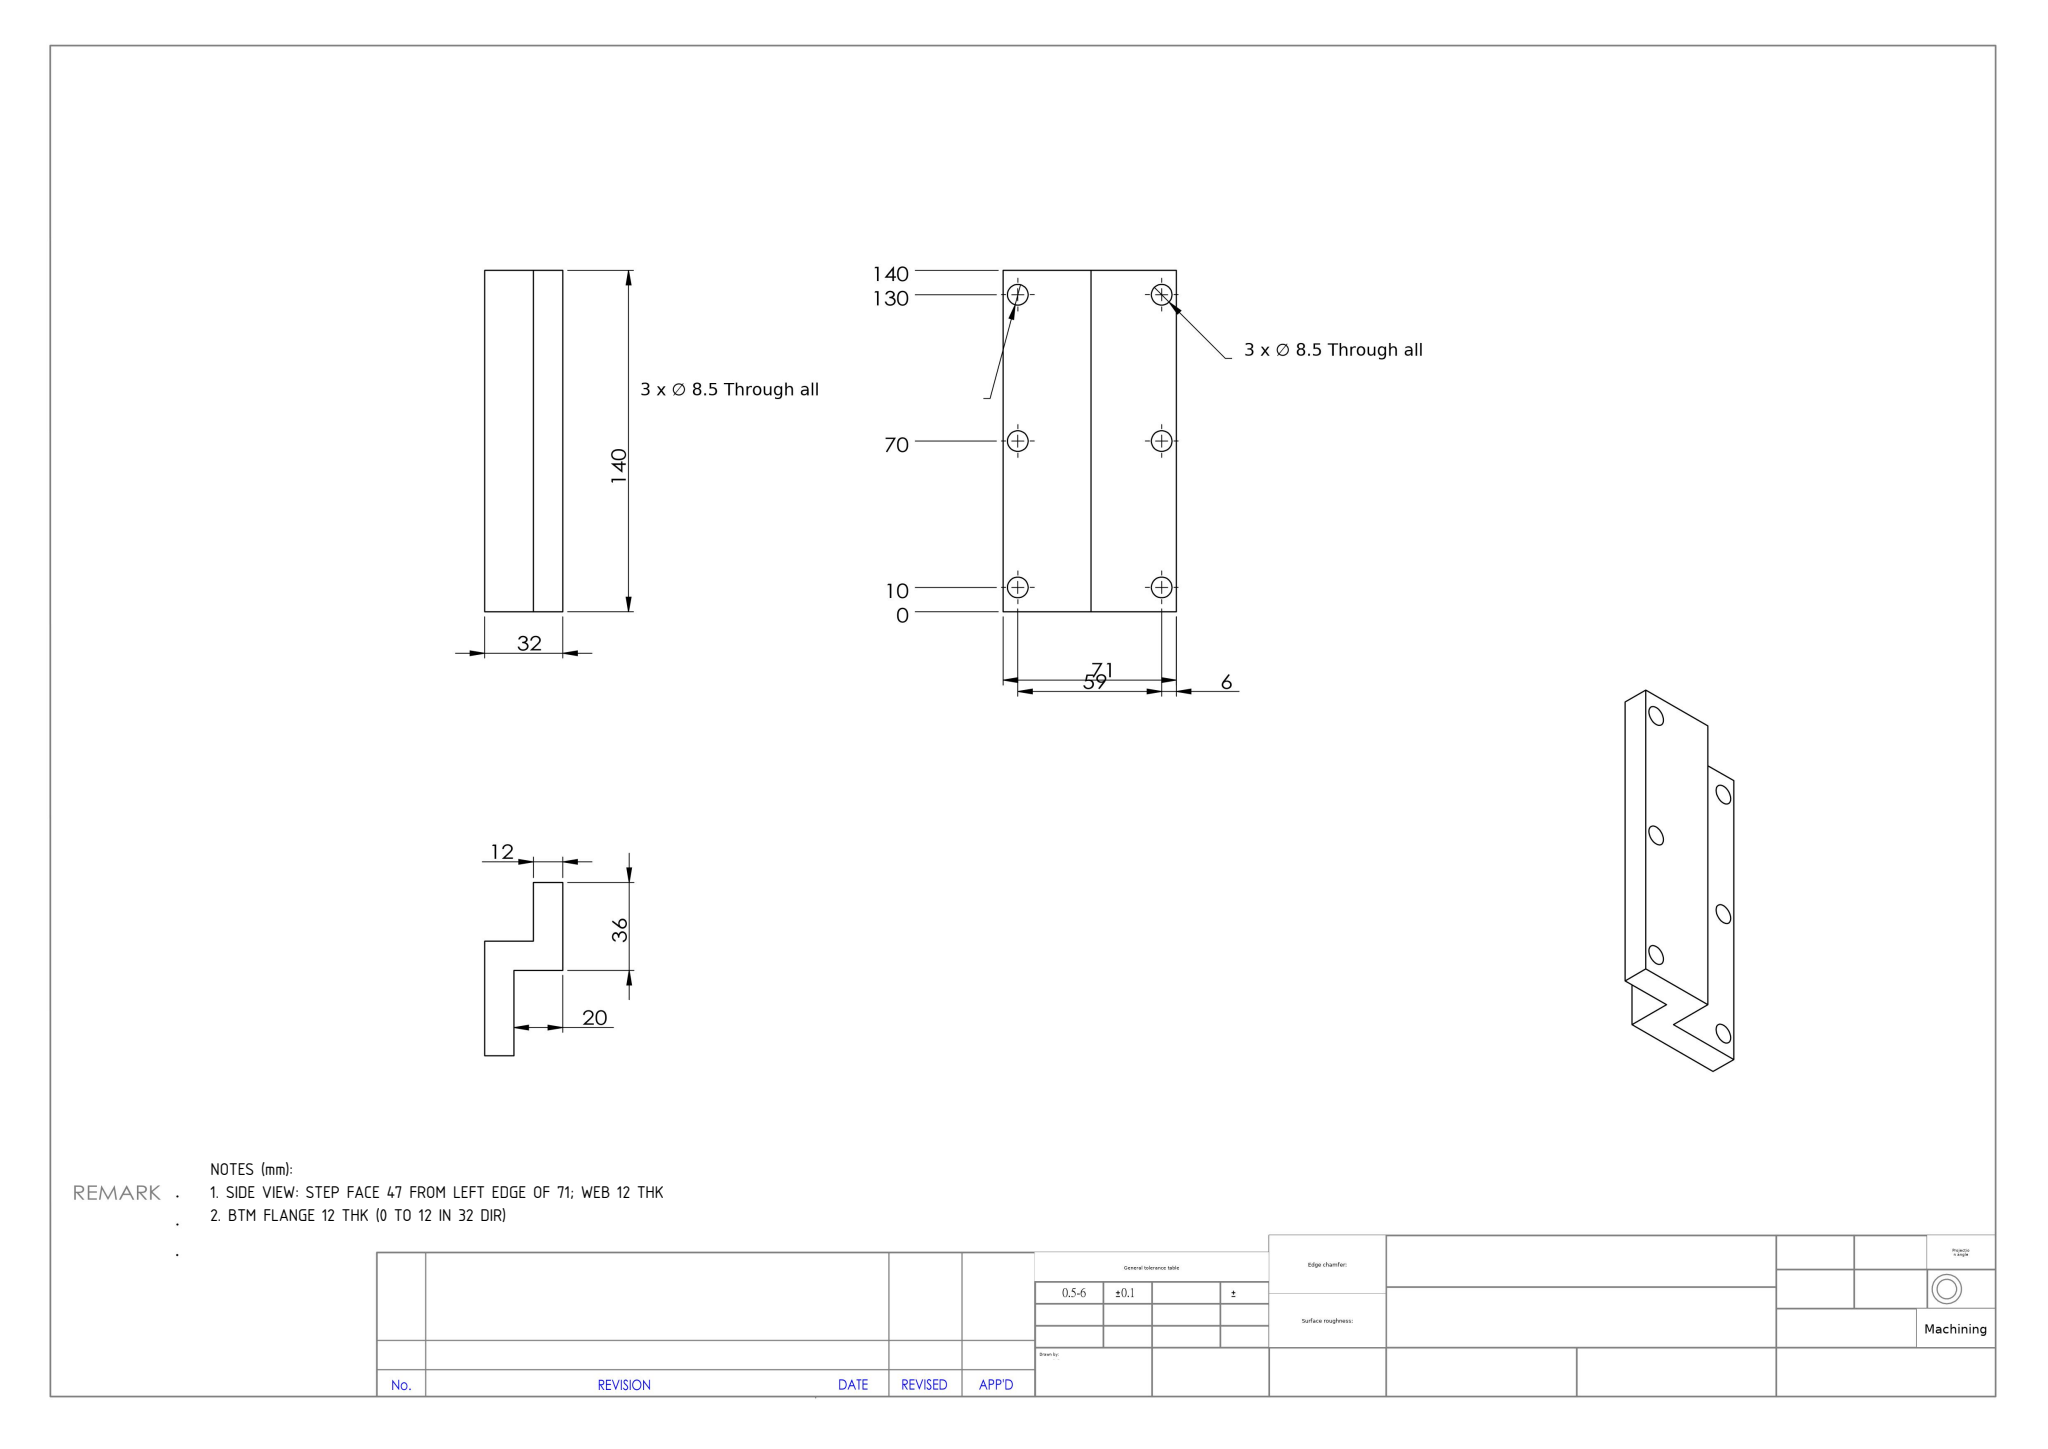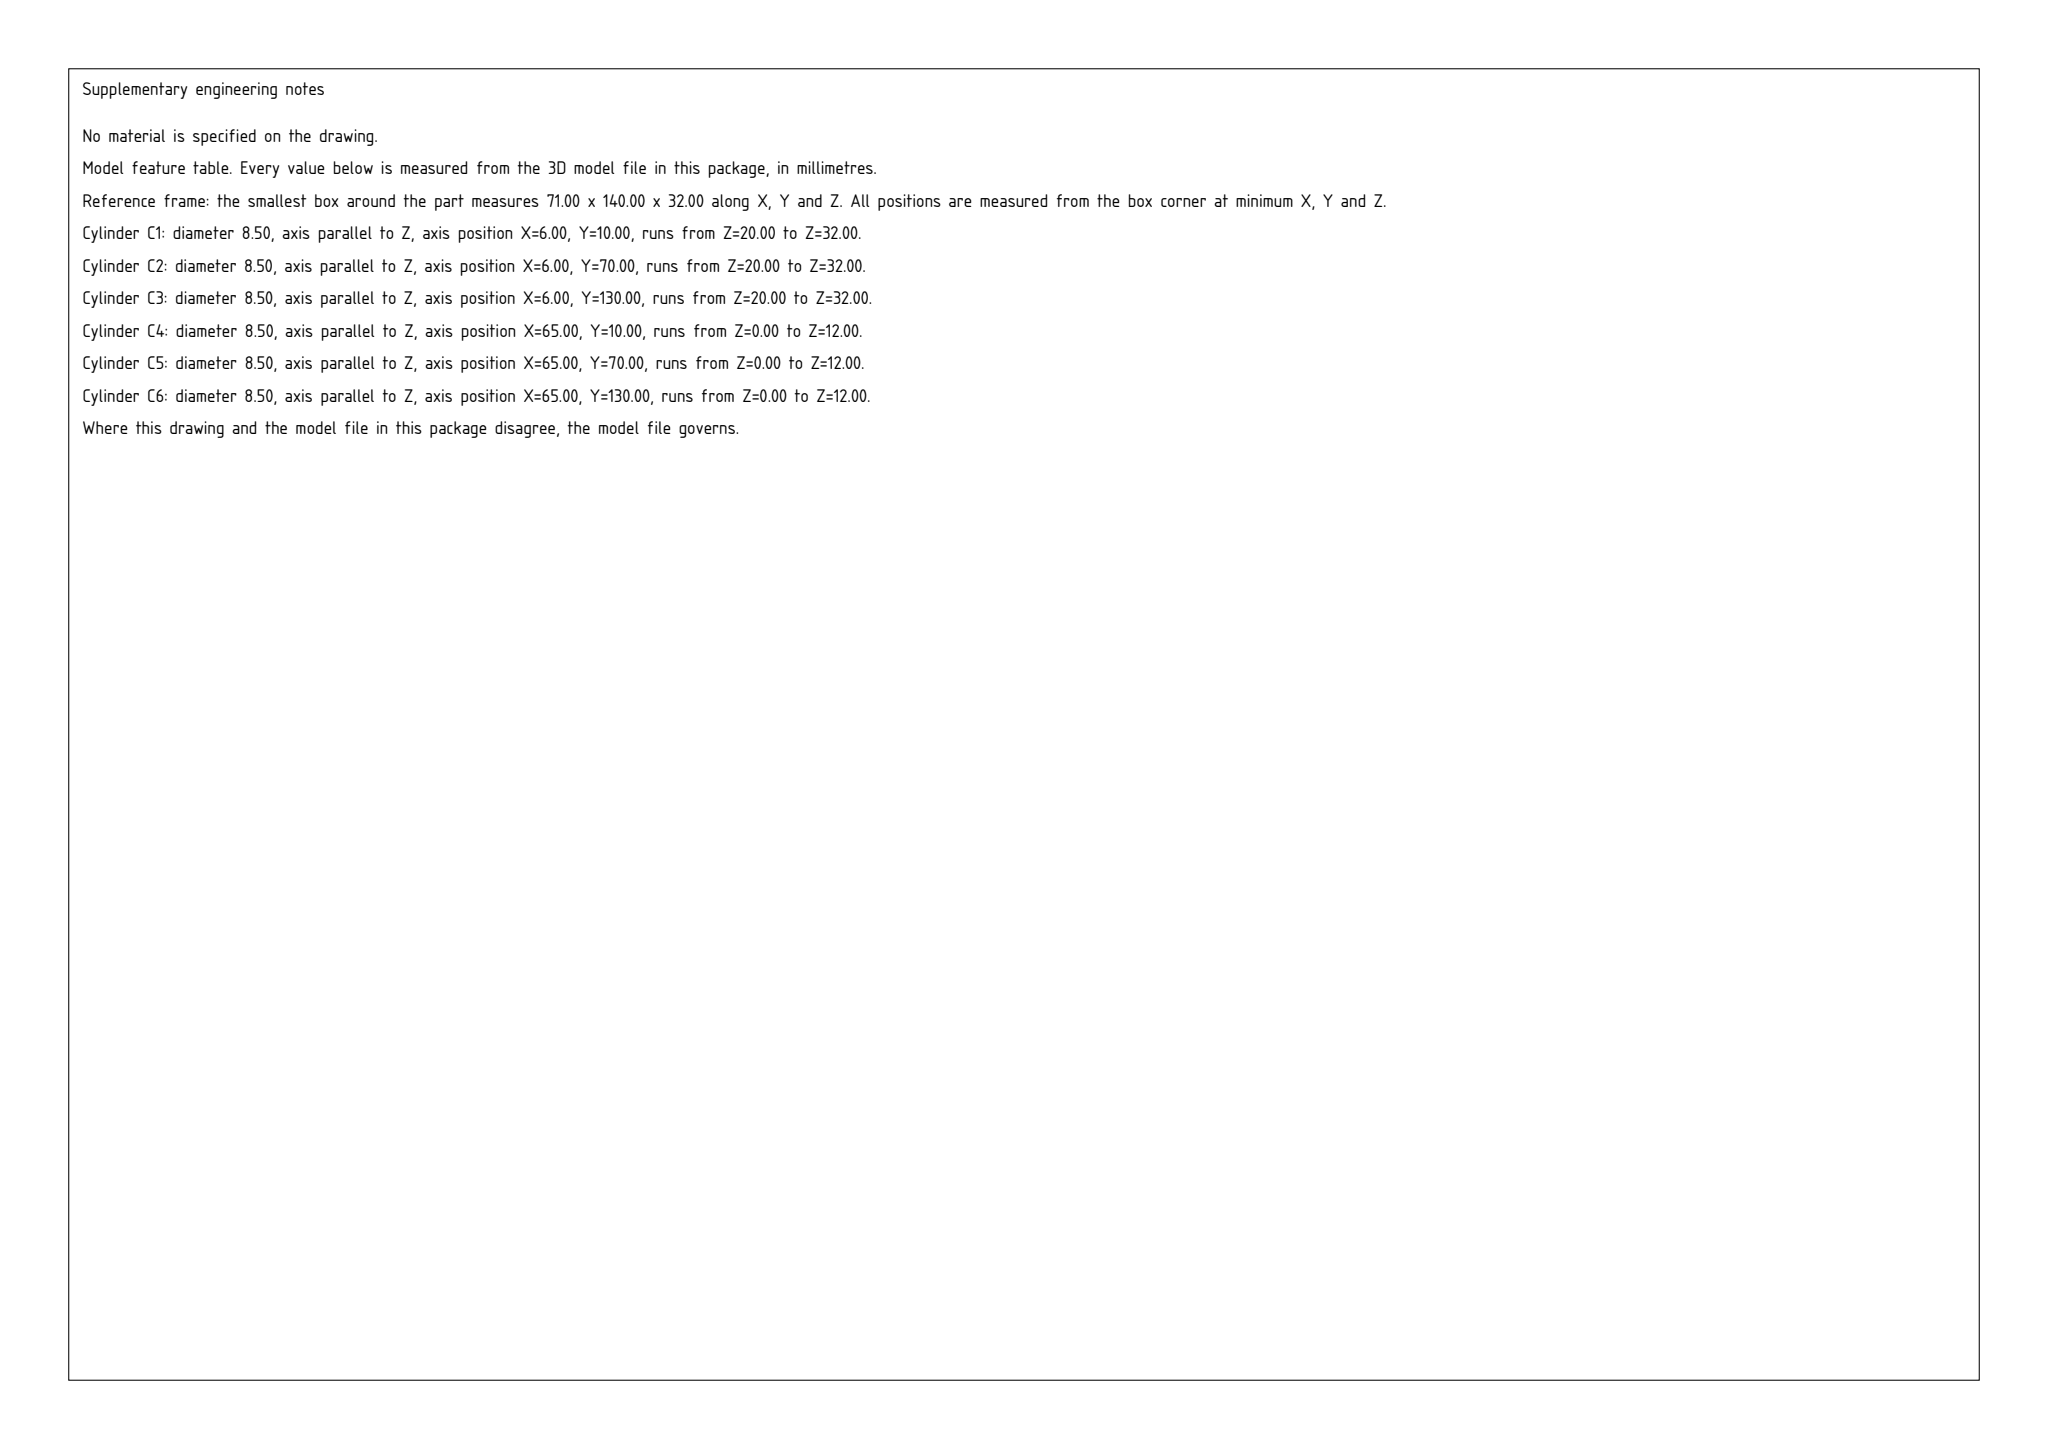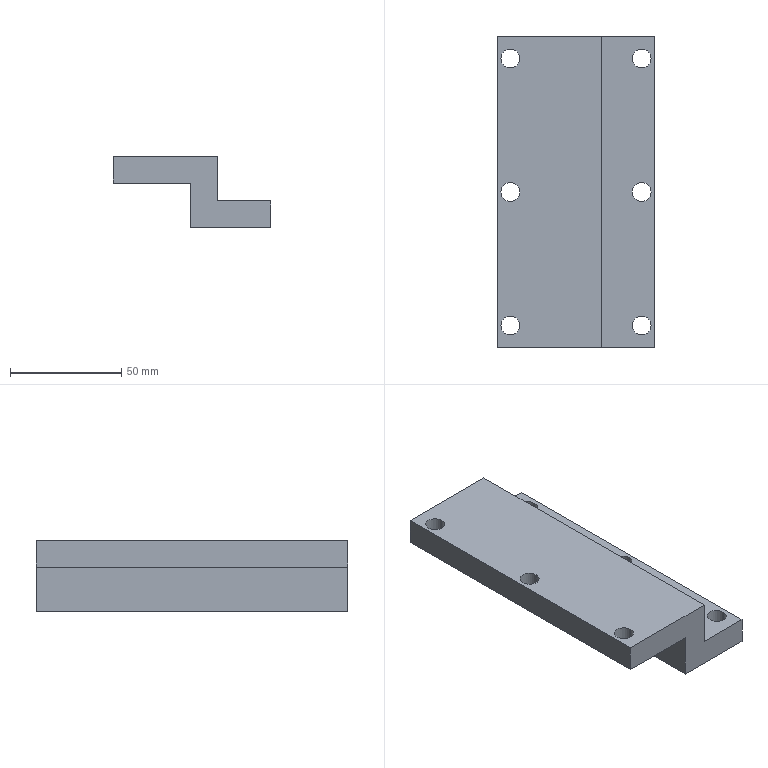Part | SolidWorks | mm | 1 solid | 22 faces | box 71 x 140 x 32 mm | volume 148794 mm3 | cylinder 12 | plane 10 | commonest cylinder face diameters 8.5 x12
Drawing notes:
SIDE VIEW: STEP FACE 47 FROM LEFT EDGE OF 71; WEB 12 THK | from the solid: axis_planes x: 0.0, 35.0, 47.0, 71.0 -> web between x35 and x47 (12 thk), lower flange face at x=47 i.e. 47 from x=0 datum used by 59/71 dims
BTM FLANGE 12 THK (0 TO 12 IN 32 DIR) | from the solid: axis_planes z: 0.0, 12.0, 20.0, 32.0 -> bottom flange spans z0-z12 = 12 thk, matching 12 upper flange and 20 step face
build123d program:
from build123d import *

# Parameters (mm, degrees)
SKETCH1_W            = 32
SKETCH1_H            = 140
BOSS_EXTRUDE1_DEPTH  = 12
SKETCH2_W            = 12
SKETCH2_H            = 140
BOSS_EXTRUDE2_DEPTH  = 24
SKETCH3_W            = 12
SKETCH3_H            = 140
BOSS_EXTRUDE3_DEPTH  = 35
M8_CLEARANCE_HOLE1_D = 8.5
M8_CLEARANCE_HOLE2_D = 8.5


with BuildPart() as part:
    # Sketch1 → Boss-Extrude1 (new body)
    with BuildSketch(Plane(origin=(0, 0, 0), x_dir=(0, 0, -1), z_dir=(1, 0, 0))):
        Rectangle(SKETCH1_W, SKETCH1_H)
    extrude(amount=BOSS_EXTRUDE1_DEPTH)

    # Sketch2 → Boss-Extrude2 (add)
    with BuildSketch(Plane(origin=(12, 0, 0), x_dir=(0, 0, -1), z_dir=(1, 0, 0))):
        with Locations((10, 0)):
            Rectangle(SKETCH2_W, SKETCH2_H)
    extrude(amount=BOSS_EXTRUDE2_DEPTH)

    # Sketch3 → Boss-Extrude3 (add)
    with BuildSketch(Plane.ZY):
        with Locations((10, 0)):
            Rectangle(SKETCH3_W, SKETCH3_H)
    extrude(amount=BOSS_EXTRUDE3_DEPTH)

    # M8 Clearance Hole1 (through all)
    with Locations(Plane(origin=(0, 0, -16), x_dir=(-1, 0, 0), z_dir=(0, 0, -1))):
        with Locations((-30, -60), (-30, 0), (-30, 60)):
            Hole(M8_CLEARANCE_HOLE1_D / 2)

    # M8 Clearance Hole2 (through all)
    with Locations(Plane(origin=(0, 0, 4), x_dir=(-1, 0, 0), z_dir=(0, 0, -1))):
        with Locations((29, 0), (29, 60), (29, -60)):
            Hole(M8_CLEARANCE_HOLE2_D / 2)


solid = part.part
STEP:
#1=CARTESIAN_POINT('',(-24.75,0.,16.));
#2=VERTEX_POINT('',#1);
#3=CARTESIAN_POINT('',(-33.25,0.,16.));
#4=VERTEX_POINT('',#3);
#5=CARTESIAN_POINT('',(-29.,0.,16.));
#6=DIRECTION('',(0.,0.,-1.));
#7=DIRECTION('',(-1.,0.,0.));
#8=AXIS2_PLACEMENT_3D('',#5,#6,#7);
#9=CIRCLE('',#8,4.25);
#10=EDGE_CURVE('',#2,#4,#9,.T.);
#11=ORIENTED_EDGE('',*,*,#10,.F.);
#12=CARTESIAN_POINT('',(-24.75,0.,4.));
#13=VERTEX_POINT('',#12);
#14=CARTESIAN_POINT('',(-24.75,0.,4.));
#15=DIRECTION('',(0.,0.,-1.));
#16=VECTOR('',#15,1000.);
#17=LINE('',#14,#16);
#18=EDGE_CURVE('',#2,#13,#17,.T.);
#19=ORIENTED_EDGE('',*,*,#18,.T.);
#20=CARTESIAN_POINT('',(-33.25,0.,4.));
#21=VERTEX_POINT('',#20);
#22=CARTESIAN_POINT('',(-29.,0.,4.));
#23=DIRECTION('',(0.,0.,-1.));
#24=DIRECTION('',(-1.,0.,0.));
#25=AXIS2_PLACEMENT_3D('',#22,#23,#24);
#26=CIRCLE('',#25,4.25);
#27=EDGE_CURVE('',#13,#21,#26,.T.);
#28=ORIENTED_EDGE('',*,*,#27,.T.);
#29=CARTESIAN_POINT('',(-33.25,0.,4.));
#30=DIRECTION('',(0.,0.,-1.));
#31=VECTOR('',#30,1000.);
#32=LINE('',#29,#31);
#33=EDGE_CURVE('',#4,#21,#32,.T.);
#34=ORIENTED_EDGE('',*,*,#33,.F.);
#35=EDGE_LOOP('',(#11,#19,#28,#34));
#36=FACE_OUTER_BOUND('',#35,.T.);
#37=CARTESIAN_POINT('',(-29.,0.,4.));
#38=DIRECTION('',(0.,0.,-1.));
#39=DIRECTION('',(-1.,0.,0.));
#40=AXIS2_PLACEMENT_3D('',#37,#38,#39);
#41=CYLINDRICAL_SURFACE('',#40,4.25);
#42=ADVANCED_FACE('',(#36),#41,.F.);
#43=CARTESIAN_POINT('',(-24.75,60.,16.));
#44=VERTEX_POINT('',#43);
#45=CARTESIAN_POINT('',(-33.25,60.,16.));
#46=VERTEX_POINT('',#45);
#47=CARTESIAN_POINT('',(-29.,60.,16.));
#48=DIRECTION('',(0.,0.,-1.));
#49=DIRECTION('',(-1.,0.,0.));
#50=AXIS2_PLACEMENT_3D('',#47,#48,#49);
#51=CIRCLE('',#50,4.25);
#52=EDGE_CURVE('',#44,#46,#51,.T.);
#53=ORIENTED_EDGE('',*,*,#52,.F.);
#54=CARTESIAN_POINT('',(-24.75,60.,4.));
#55=VERTEX_POINT('',#54);
#56=CARTESIAN_POINT('',(-24.75,60.,4.));
#57=DIRECTION('',(0.,0.,-1.));
#58=VECTOR('',#57,1000.);
#59=LINE('',#56,#58);
#60=EDGE_CURVE('',#44,#55,#59,.T.);
#61=ORIENTED_EDGE('',*,*,#60,.T.);
#62=CARTESIAN_POINT('',(-33.25,60.,4.));
#63=VERTEX_POINT('',#62);
#64=CARTESIAN_POINT('',(-29.,60.,4.));
#65=DIRECTION('',(0.,0.,-1.));
#66=DIRECTION('',(-1.,0.,0.));
#67=AXIS2_PLACEMENT_3D('',#64,#65,#66);
#68=CIRCLE('',#67,4.25);
#69=EDGE_CURVE('',#55,#63,#68,.T.);
#70=ORIENTED_EDGE('',*,*,#69,.T.);
#71=CARTESIAN_POINT('',(-33.25,60.,4.));
#72=DIRECTION('',(0.,0.,-1.));
#73=VECTOR('',#72,1000.);
#74=LINE('',#71,#73);
#75=EDGE_CURVE('',#46,#63,#74,.T.);
#76=ORIENTED_EDGE('',*,*,#75,.F.);
#77=EDGE_LOOP('',(#53,#61,#70,#76));
#78=FACE_OUTER_BOUND('',#77,.T.);
#79=CARTESIAN_POINT('',(-29.,60.,4.));
#80=DIRECTION('',(0.,0.,-1.));
#81=DIRECTION('',(-1.,0.,0.));
#82=AXIS2_PLACEMENT_3D('',#79,#80,#81);
#83=CYLINDRICAL_SURFACE('',#82,4.25);
#84=ADVANCED_FACE('',(#78),#83,.F.);
#85=CARTESIAN_POINT('',(-24.75,-60.,16.));
#86=VERTEX_POINT('',#85);
#87=CARTESIAN_POINT('',(-33.25,-60.,16.));
#88=VERTEX_POINT('',#87);
#89=CARTESIAN_POINT('',(-29.,-60.,16.));
#90=DIRECTION('',(0.,0.,-1.));
#91=DIRECTION('',(-1.,0.,0.));
#92=AXIS2_PLACEMENT_3D('',#89,#90,#91);
#93=CIRCLE('',#92,4.25);
#94=EDGE_CURVE('',#86,#88,#93,.T.);
#95=ORIENTED_EDGE('',*,*,#94,.F.);
#96=CARTESIAN_POINT('',(-24.75,-60.,4.));
#97=VERTEX_POINT('',#96);
#98=CARTESIAN_POINT('',(-24.75,-60.,4.));
#99=DIRECTION('',(0.,0.,-1.));
#100=VECTOR('',#99,1000.);
#101=LINE('',#98,#100);
#102=EDGE_CURVE('',#86,#97,#101,.T.);
#103=ORIENTED_EDGE('',*,*,#102,.T.);
#104=CARTESIAN_POINT('',(-33.25,-60.,4.));
#105=VERTEX_POINT('',#104);
#106=CARTESIAN_POINT('',(-29.,-60.,4.));
#107=DIRECTION('',(0.,0.,-1.));
#108=DIRECTION('',(-1.,0.,0.));
#109=AXIS2_PLACEMENT_3D('',#106,#107,#108);
#110=CIRCLE('',#109,4.25);
#111=EDGE_CURVE('',#97,#105,#110,.T.);
#112=ORIENTED_EDGE('',*,*,#111,.T.);
#113=CARTESIAN_POINT('',(-33.25,-60.,4.));
#114=DIRECTION('',(0.,0.,-1.));
#115=VECTOR('',#114,1000.);
#116=LINE('',#113,#115);
#117=EDGE_CURVE('',#88,#105,#116,.T.);
#118=ORIENTED_EDGE('',*,*,#117,.F.);
#119=EDGE_LOOP('',(#95,#103,#112,#118));
#120=FACE_OUTER_BOUND('',#119,.T.);
#121=CARTESIAN_POINT('',(-29.,-60.,4.));
#122=DIRECTION('',(0.,0.,-1.));
#123=DIRECTION('',(-1.,0.,0.));
#124=AXIS2_PLACEMENT_3D('',#121,#122,#123);
#125=CYLINDRICAL_SURFACE('',#124,4.25);
#126=ADVANCED_FACE('',(#120),#125,.F.);
#127=CARTESIAN_POINT('',(34.25,0.,-4.));
#128=VERTEX_POINT('',#127);
#129=CARTESIAN_POINT('',(25.75,0.,-4.));
#130=VERTEX_POINT('',#129);
#131=CARTESIAN_POINT('',(30.,0.,-4.));
#132=DIRECTION('',(0.,0.,-1.));
#133=DIRECTION('',(0.,1.,0.));
#134=AXIS2_PLACEMENT_3D('',#131,#132,#133);
#135=CIRCLE('',#134,4.25);
#136=EDGE_CURVE('',#128,#130,#135,.T.);
#137=ORIENTED_EDGE('',*,*,#136,.F.);
#138=CARTESIAN_POINT('',(34.25,0.,-16.));
#139=VERTEX_POINT('',#138);
#140=CARTESIAN_POINT('',(34.25,0.,-16.));
#141=DIRECTION('',(0.,0.,-1.));
#142=VECTOR('',#141,1000.);
#143=LINE('',#140,#142);
#144=EDGE_CURVE('',#128,#139,#143,.T.);
#145=ORIENTED_EDGE('',*,*,#144,.T.);
#146=CARTESIAN_POINT('',(25.75,0.,-16.));
#147=VERTEX_POINT('',#146);
#148=CARTESIAN_POINT('',(30.,0.,-16.));
#149=DIRECTION('',(0.,0.,-1.));
#150=DIRECTION('',(-1.,0.,0.));
#151=AXIS2_PLACEMENT_3D('',#148,#149,#150);
#152=CIRCLE('',#151,4.25);
#153=EDGE_CURVE('',#139,#147,#152,.T.);
#154=ORIENTED_EDGE('',*,*,#153,.T.);
#155=CARTESIAN_POINT('',(25.75,0.,-16.));
#156=DIRECTION('',(0.,0.,-1.));
#157=VECTOR('',#156,1000.);
#158=LINE('',#155,#157);
#159=EDGE_CURVE('',#130,#147,#158,.T.);
#160=ORIENTED_EDGE('',*,*,#159,.F.);
#161=EDGE_LOOP('',(#137,#145,#154,#160));
#162=FACE_OUTER_BOUND('',#161,.T.);
#163=CARTESIAN_POINT('',(30.,0.,-16.));
#164=DIRECTION('',(0.,0.,-1.));
#165=DIRECTION('',(-1.,0.,0.));
#166=AXIS2_PLACEMENT_3D('',#163,#164,#165);
#167=CYLINDRICAL_SURFACE('',#166,4.25);
#168=ADVANCED_FACE('',(#162),#167,.F.);
#169=CARTESIAN_POINT('',(34.25,60.,-4.));
#170=VERTEX_POINT('',#169);
#171=CARTESIAN_POINT('',(25.75,60.,-4.));
#172=VERTEX_POINT('',#171);
#173=CARTESIAN_POINT('',(30.,60.,-4.));
#174=DIRECTION('',(0.,0.,-1.));
#175=DIRECTION('',(0.,1.,0.));
#176=AXIS2_PLACEMENT_3D('',#173,#174,#175);
#177=CIRCLE('',#176,4.25);
#178=EDGE_CURVE('',#170,#172,#177,.T.);
#179=ORIENTED_EDGE('',*,*,#178,.F.);
#180=CARTESIAN_POINT('',(34.25,60.,-16.));
#181=VERTEX_POINT('',#180);
#182=CARTESIAN_POINT('',(34.25,60.,-16.));
#183=DIRECTION('',(0.,0.,-1.));
#184=VECTOR('',#183,1000.);
#185=LINE('',#182,#184);
#186=EDGE_CURVE('',#170,#181,#185,.T.);
#187=ORIENTED_EDGE('',*,*,#186,.T.);
#188=CARTESIAN_POINT('',(25.75,60.,-16.));
#189=VERTEX_POINT('',#188);
#190=CARTESIAN_POINT('',(30.,60.,-16.));
#191=DIRECTION('',(0.,0.,-1.));
#192=DIRECTION('',(-1.,0.,0.));
#193=AXIS2_PLACEMENT_3D('',#190,#191,#192);
#194=CIRCLE('',#193,4.25);
#195=EDGE_CURVE('',#181,#189,#194,.T.);
#196=ORIENTED_EDGE('',*,*,#195,.T.);
#197=CARTESIAN_POINT('',(25.75,60.,-16.));
#198=DIRECTION('',(0.,0.,-1.));
#199=VECTOR('',#198,1000.);
#200=LINE('',#197,#199);
#201=EDGE_CURVE('',#172,#189,#200,.T.);
#202=ORIENTED_EDGE('',*,*,#201,.F.);
#203=EDGE_LOOP('',(#179,#187,#196,#202));
#204=FACE_OUTER_BOUND('',#203,.T.);
#205=CARTESIAN_POINT('',(30.,60.,-16.));
#206=DIRECTION('',(0.,0.,-1.));
#207=DIRECTION('',(-1.,0.,0.));
#208=AXIS2_PLACEMENT_3D('',#205,#206,#207);
#209=CYLINDRICAL_SURFACE('',#208,4.25);
#210=ADVANCED_FACE('',(#204),#209,.F.);
#211=CARTESIAN_POINT('',(34.25,-60.,-4.));
#212=VERTEX_POINT('',#211);
#213=CARTESIAN_POINT('',(25.75,-60.,-4.));
#214=VERTEX_POINT('',#213);
#215=CARTESIAN_POINT('',(30.,-60.,-4.));
#216=DIRECTION('',(0.,0.,-1.));
#217=DIRECTION('',(0.,1.,0.));
#218=AXIS2_PLACEMENT_3D('',#215,#216,#217);
#219=CIRCLE('',#218,4.25);
#220=EDGE_CURVE('',#212,#214,#219,.T.);
#221=ORIENTED_EDGE('',*,*,#220,.F.);
#222=CARTESIAN_POINT('',(34.25,-60.,-16.));
#223=VERTEX_POINT('',#222);
#224=CARTESIAN_POINT('',(34.25,-60.,-16.));
#225=DIRECTION('',(0.,0.,-1.));
#226=VECTOR('',#225,1000.);
#227=LINE('',#224,#226);
#228=EDGE_CURVE('',#212,#223,#227,.T.);
#229=ORIENTED_EDGE('',*,*,#228,.T.);
#230=CARTESIAN_POINT('',(25.75,-60.,-16.));
#231=VERTEX_POINT('',#230);
#232=CARTESIAN_POINT('',(30.,-60.,-16.));
#233=DIRECTION('',(0.,0.,-1.));
#234=DIRECTION('',(-1.,0.,0.));
#235=AXIS2_PLACEMENT_3D('',#232,#233,#234);
#236=CIRCLE('',#235,4.25);
#237=EDGE_CURVE('',#223,#231,#236,.T.);
#238=ORIENTED_EDGE('',*,*,#237,.T.);
#239=CARTESIAN_POINT('',(25.75,-60.,-16.));
#240=DIRECTION('',(0.,0.,-1.));
#241=VECTOR('',#240,1000.);
#242=LINE('',#239,#241);
#243=EDGE_CURVE('',#214,#231,#242,.T.);
#244=ORIENTED_EDGE('',*,*,#243,.F.);
#245=EDGE_LOOP('',(#221,#229,#238,#244));
#246=FACE_OUTER_BOUND('',#245,.T.);
#247=CARTESIAN_POINT('',(30.,-60.,-16.));
#248=DIRECTION('',(0.,0.,-1.));
#249=DIRECTION('',(-1.,0.,0.));
#250=AXIS2_PLACEMENT_3D('',#247,#248,#249);
#251=CYLINDRICAL_SURFACE('',#250,4.25);
#252=ADVANCED_FACE('',(#246),#251,.F.);
#253=CARTESIAN_POINT('',(12.,70.,-4.));
#254=VERTEX_POINT('',#253);
#255=CARTESIAN_POINT('',(12.,-70.,-4.));
#256=VERTEX_POINT('',#255);
#257=CARTESIAN_POINT('',(12.,70.,-4.));
#258=DIRECTION('',(0.,-1.,-0.));
#259=VECTOR('',#258,1000.);
#260=LINE('',#257,#259);
#261=EDGE_CURVE('',#254,#256,#260,.T.);
#262=ORIENTED_EDGE('',*,*,#261,.F.);
#263=CARTESIAN_POINT('',(12.,70.,16.));
#264=VERTEX_POINT('',#263);
#265=CARTESIAN_POINT('',(12.,70.,16.));
#266=DIRECTION('',(0.,0.,1.));
#267=VECTOR('',#266,1000.);
#268=LINE('',#265,#267);
#269=EDGE_CURVE('',#254,#264,#268,.T.);
#270=ORIENTED_EDGE('',*,*,#269,.T.);
#271=CARTESIAN_POINT('',(12.,-70.,16.));
#272=VERTEX_POINT('',#271);
#273=CARTESIAN_POINT('',(12.,-70.,16.));
#274=DIRECTION('',(0.,-1.,0.));
#275=VECTOR('',#274,1000.);
#276=LINE('',#273,#275);
#277=EDGE_CURVE('',#264,#272,#276,.T.);
#278=ORIENTED_EDGE('',*,*,#277,.T.);
#279=CARTESIAN_POINT('',(12.,-70.,16.));
#280=DIRECTION('',(0.,0.,-1.));
#281=VECTOR('',#280,1000.);
#282=LINE('',#279,#281);
#283=EDGE_CURVE('',#272,#256,#282,.T.);
#284=ORIENTED_EDGE('',*,*,#283,.T.);
#285=EDGE_LOOP('',(#262,#270,#278,#284));
#286=FACE_OUTER_BOUND('',#285,.T.);
#287=CARTESIAN_POINT('',(12.,0.,0.));
#288=DIRECTION('',(-1.,0.,0.));
#289=DIRECTION('',(0.,0.,1.));
#290=AXIS2_PLACEMENT_3D('',#287,#288,#289);
#291=PLANE('',#290);
#292=ADVANCED_FACE('',(#286),#291,.F.);
#293=CARTESIAN_POINT('',(30.,0.,-16.));
#294=DIRECTION('',(0.,0.,-1.));
#295=DIRECTION('',(-1.,0.,0.));
#296=AXIS2_PLACEMENT_3D('',#293,#294,#295);
#297=CIRCLE('',#296,4.25);
#298=EDGE_CURVE('',#147,#139,#297,.T.);
#299=ORIENTED_EDGE('',*,*,#298,.F.);
#300=ORIENTED_EDGE('',*,*,#153,.F.);
#301=EDGE_LOOP('',(#299,#300));
#302=FACE_BOUND('',#301,.T.);
#303=CARTESIAN_POINT('',(30.,60.,-16.));
#304=DIRECTION('',(0.,0.,-1.));
#305=DIRECTION('',(-1.,0.,0.));
#306=AXIS2_PLACEMENT_3D('',#303,#304,#305);
#307=CIRCLE('',#306,4.25);
#308=EDGE_CURVE('',#189,#181,#307,.T.);
#309=ORIENTED_EDGE('',*,*,#308,.F.);
#310=ORIENTED_EDGE('',*,*,#195,.F.);
#311=EDGE_LOOP('',(#309,#310));
#312=FACE_BOUND('',#311,.T.);
#313=CARTESIAN_POINT('',(30.,-60.,-16.));
#314=DIRECTION('',(0.,0.,-1.));
#315=DIRECTION('',(-1.,0.,0.));
#316=AXIS2_PLACEMENT_3D('',#313,#314,#315);
#317=CIRCLE('',#316,4.25);
#318=EDGE_CURVE('',#231,#223,#317,.T.);
#319=ORIENTED_EDGE('',*,*,#318,.F.);
#320=ORIENTED_EDGE('',*,*,#237,.F.);
#321=EDGE_LOOP('',(#319,#320));
#322=FACE_BOUND('',#321,.T.);
#323=CARTESIAN_POINT('',(0.,-70.,-16.));
#324=VERTEX_POINT('',#323);
#325=CARTESIAN_POINT('',(0.,70.,-16.));
#326=VERTEX_POINT('',#325);
#327=CARTESIAN_POINT('',(0.,-70.,-16.));
#328=DIRECTION('',(0.,1.,0.));
#329=VECTOR('',#328,1000.);
#330=LINE('',#327,#329);
#331=EDGE_CURVE('',#324,#326,#330,.T.);
#332=ORIENTED_EDGE('',*,*,#331,.T.);
#333=CARTESIAN_POINT('',(36.,70.,-16.));
#334=VERTEX_POINT('',#333);
#335=CARTESIAN_POINT('',(12.,70.,-16.));
#336=DIRECTION('',(-1.,0.,0.));
#337=VECTOR('',#336,1000.);
#338=LINE('',#335,#337);
#339=EDGE_CURVE('',#334,#326,#338,.T.);
#340=ORIENTED_EDGE('',*,*,#339,.F.);
#341=CARTESIAN_POINT('',(36.,-70.,-16.));
#342=VERTEX_POINT('',#341);
#343=CARTESIAN_POINT('',(36.,70.,-16.));
#344=DIRECTION('',(0.,1.,0.));
#345=VECTOR('',#344,1000.);
#346=LINE('',#343,#345);
#347=EDGE_CURVE('',#342,#334,#346,.T.);
#348=ORIENTED_EDGE('',*,*,#347,.F.);
#349=CARTESIAN_POINT('',(12.,-70.,-16.));
#350=DIRECTION('',(-1.,0.,0.));
#351=VECTOR('',#350,1000.);
#352=LINE('',#349,#351);
#353=EDGE_CURVE('',#342,#324,#352,.T.);
#354=ORIENTED_EDGE('',*,*,#353,.T.);
#355=EDGE_LOOP('',(#332,#340,#348,#354));
#356=FACE_OUTER_BOUND('',#355,.T.);
#357=CARTESIAN_POINT('',(12.,-70.,-16.));
#358=DIRECTION('',(0.,0.,1.));
#359=DIRECTION('',(1.,0.,0.));
#360=AXIS2_PLACEMENT_3D('',#357,#358,#359);
#361=PLANE('',#360);
#362=ADVANCED_FACE('',(#302,#312,#322,#356),#361,.F.);
#363=CARTESIAN_POINT('',(0.,70.,4.));
#364=VERTEX_POINT('',#363);
#365=CARTESIAN_POINT('',(0.,70.,16.));
#366=DIRECTION('',(0.,0.,1.));
#367=VECTOR('',#366,1000.);
#368=LINE('',#365,#367);
#369=EDGE_CURVE('',#326,#364,#368,.T.);
#370=ORIENTED_EDGE('',*,*,#369,.T.);
#371=CARTESIAN_POINT('',(-35.,70.,4.));
#372=VERTEX_POINT('',#371);
#373=CARTESIAN_POINT('',(-35.,70.,4.));
#374=DIRECTION('',(1.,0.,0.));
#375=VECTOR('',#374,1000.);
#376=LINE('',#373,#375);
#377=EDGE_CURVE('',#372,#364,#376,.T.);
#378=ORIENTED_EDGE('',*,*,#377,.F.);
#379=CARTESIAN_POINT('',(-35.,70.,16.));
#380=VERTEX_POINT('',#379);
#381=CARTESIAN_POINT('',(-35.,70.,16.));
#382=DIRECTION('',(0.,0.,-1.));
#383=VECTOR('',#382,1000.);
#384=LINE('',#381,#383);
#385=EDGE_CURVE('',#380,#372,#384,.T.);
#386=ORIENTED_EDGE('',*,*,#385,.F.);
#387=CARTESIAN_POINT('',(12.,70.,16.));
#388=DIRECTION('',(-1.,0.,0.));
#389=VECTOR('',#388,1000.);
#390=LINE('',#387,#389);
#391=EDGE_CURVE('',#264,#380,#390,.T.);
#392=ORIENTED_EDGE('',*,*,#391,.F.);
#393=ORIENTED_EDGE('',*,*,#269,.F.);
#394=CARTESIAN_POINT('',(36.,70.,-4.));
#395=VERTEX_POINT('',#394);
#396=CARTESIAN_POINT('',(36.,70.,-4.));
#397=DIRECTION('',(-1.,0.,0.));
#398=VECTOR('',#397,1000.);
#399=LINE('',#396,#398);
#400=EDGE_CURVE('',#395,#254,#399,.T.);
#401=ORIENTED_EDGE('',*,*,#400,.F.);
#402=CARTESIAN_POINT('',(36.,70.,-16.));
#403=DIRECTION('',(0.,0.,1.));
#404=VECTOR('',#403,1000.);
#405=LINE('',#402,#404);
#406=EDGE_CURVE('',#334,#395,#405,.T.);
#407=ORIENTED_EDGE('',*,*,#406,.F.);
#408=ORIENTED_EDGE('',*,*,#339,.T.);
#409=EDGE_LOOP('',(#370,#378,#386,#392,#393,#401,#407,#408));
#410=FACE_OUTER_BOUND('',#409,.T.);
#411=CARTESIAN_POINT('',(12.,70.,16.));
#412=DIRECTION('',(0.,-1.,0.));
#413=DIRECTION('',(0.,0.,-1.));
#414=AXIS2_PLACEMENT_3D('',#411,#412,#413);
#415=PLANE('',#414);
#416=ADVANCED_FACE('',(#410),#415,.F.);
#417=CARTESIAN_POINT('',(-29.,0.,16.));
#418=DIRECTION('',(0.,0.,-1.));
#419=DIRECTION('',(-1.,0.,0.));
#420=AXIS2_PLACEMENT_3D('',#417,#418,#419);
#421=CIRCLE('',#420,4.25);
#422=EDGE_CURVE('',#4,#2,#421,.T.);
#423=ORIENTED_EDGE('',*,*,#422,.T.);
#424=ORIENTED_EDGE('',*,*,#10,.T.);
#425=EDGE_LOOP('',(#423,#424));
#426=FACE_BOUND('',#425,.T.);
#427=CARTESIAN_POINT('',(-29.,60.,16.));
#428=DIRECTION('',(0.,0.,-1.));
#429=DIRECTION('',(-1.,0.,0.));
#430=AXIS2_PLACEMENT_3D('',#427,#428,#429);
#431=CIRCLE('',#430,4.25);
#432=EDGE_CURVE('',#46,#44,#431,.T.);
#433=ORIENTED_EDGE('',*,*,#432,.T.);
#434=ORIENTED_EDGE('',*,*,#52,.T.);
#435=EDGE_LOOP('',(#433,#434));
#436=FACE_BOUND('',#435,.T.);
#437=CARTESIAN_POINT('',(-29.,-60.,16.));
#438=DIRECTION('',(0.,0.,-1.));
#439=DIRECTION('',(-1.,0.,0.));
#440=AXIS2_PLACEMENT_3D('',#437,#438,#439);
#441=CIRCLE('',#440,4.25);
#442=EDGE_CURVE('',#88,#86,#441,.T.);
#443=ORIENTED_EDGE('',*,*,#442,.T.);
#444=ORIENTED_EDGE('',*,*,#94,.T.);
#445=EDGE_LOOP('',(#443,#444));
#446=FACE_BOUND('',#445,.T.);
#447=ORIENTED_EDGE('',*,*,#391,.T.);
#448=CARTESIAN_POINT('',(-35.,-70.,16.));
#449=VERTEX_POINT('',#448);
#450=CARTESIAN_POINT('',(-35.,-70.,16.));
#451=DIRECTION('',(0.,1.,0.));
#452=VECTOR('',#451,1000.);
#453=LINE('',#450,#452);
#454=EDGE_CURVE('',#449,#380,#453,.T.);
#455=ORIENTED_EDGE('',*,*,#454,.F.);
#456=CARTESIAN_POINT('',(12.,-70.,16.));
#457=DIRECTION('',(-1.,0.,0.));
#458=VECTOR('',#457,1000.);
#459=LINE('',#456,#458);
#460=EDGE_CURVE('',#272,#449,#459,.T.);
#461=ORIENTED_EDGE('',*,*,#460,.F.);
#462=ORIENTED_EDGE('',*,*,#277,.F.);
#463=EDGE_LOOP('',(#447,#455,#461,#462));
#464=FACE_OUTER_BOUND('',#463,.T.);
#465=CARTESIAN_POINT('',(12.,-70.,16.));
#466=DIRECTION('',(0.,0.,-1.));
#467=DIRECTION('',(-1.,0.,0.));
#468=AXIS2_PLACEMENT_3D('',#465,#466,#467);
#469=PLANE('',#468);
#470=ADVANCED_FACE('',(#426,#436,#446,#464),#469,.F.);
#471=ORIENTED_EDGE('',*,*,#460,.T.);
#472=CARTESIAN_POINT('',(-35.,-70.,4.));
#473=VERTEX_POINT('',#472);
#474=CARTESIAN_POINT('',(-35.,-70.,16.));
#475=DIRECTION('',(0.,0.,1.));
#476=VECTOR('',#475,1000.);
#477=LINE('',#474,#476);
#478=EDGE_CURVE('',#473,#449,#477,.T.);
#479=ORIENTED_EDGE('',*,*,#478,.F.);
#480=CARTESIAN_POINT('',(0.,-70.,4.));
#481=VERTEX_POINT('',#480);
#482=CARTESIAN_POINT('',(-35.,-70.,4.));
#483=DIRECTION('',(1.,0.,0.));
#484=VECTOR('',#483,1000.);
#485=LINE('',#482,#484);
#486=EDGE_CURVE('',#473,#481,#485,.T.);
#487=ORIENTED_EDGE('',*,*,#486,.T.);
#488=CARTESIAN_POINT('',(0.,-70.,16.));
#489=DIRECTION('',(0.,0.,-1.));
#490=VECTOR('',#489,1000.);
#491=LINE('',#488,#490);
#492=EDGE_CURVE('',#481,#324,#491,.T.);
#493=ORIENTED_EDGE('',*,*,#492,.T.);
#494=ORIENTED_EDGE('',*,*,#353,.F.);
#495=CARTESIAN_POINT('',(36.,-70.,-4.));
#496=VERTEX_POINT('',#495);
#497=CARTESIAN_POINT('',(36.,-70.,-16.));
#498=DIRECTION('',(0.,0.,-1.));
#499=VECTOR('',#498,1000.);
#500=LINE('',#497,#499);
#501=EDGE_CURVE('',#496,#342,#500,.T.);
#502=ORIENTED_EDGE('',*,*,#501,.F.);
#503=CARTESIAN_POINT('',(36.,-70.,-4.));
#504=DIRECTION('',(-1.,0.,0.));
#505=VECTOR('',#504,1000.);
#506=LINE('',#503,#505);
#507=EDGE_CURVE('',#496,#256,#506,.T.);
#508=ORIENTED_EDGE('',*,*,#507,.T.);
#509=ORIENTED_EDGE('',*,*,#283,.F.);
#510=EDGE_LOOP('',(#471,#479,#487,#493,#494,#502,#508,#509));
#511=FACE_OUTER_BOUND('',#510,.T.);
#512=CARTESIAN_POINT('',(12.,-70.,16.));
#513=DIRECTION('',(0.,1.,0.));
#514=DIRECTION('',(0.,0.,1.));
#515=AXIS2_PLACEMENT_3D('',#512,#513,#514);
#516=PLANE('',#515);
#517=ADVANCED_FACE('',(#511),#516,.F.);
#518=CARTESIAN_POINT('',(0.,-70.,4.));
#519=DIRECTION('',(0.,-1.,0.));
#520=VECTOR('',#519,1000.);
#521=LINE('',#518,#520);
#522=EDGE_CURVE('',#364,#481,#521,.T.);
#523=ORIENTED_EDGE('',*,*,#522,.F.);
#524=ORIENTED_EDGE('',*,*,#369,.F.);
#525=ORIENTED_EDGE('',*,*,#331,.F.);
#526=ORIENTED_EDGE('',*,*,#492,.F.);
#527=EDGE_LOOP('',(#523,#524,#525,#526));
#528=FACE_OUTER_BOUND('',#527,.T.);
#529=CARTESIAN_POINT('',(0.,0.,0.));
#530=DIRECTION('',(-1.,0.,0.));
#531=DIRECTION('',(0.,0.,1.));
#532=AXIS2_PLACEMENT_3D('',#529,#530,#531);
#533=PLANE('',#532);
#534=ADVANCED_FACE('',(#528),#533,.T.);
#535=CARTESIAN_POINT('',(30.,0.,-4.));
#536=DIRECTION('',(0.,0.,-1.));
#537=DIRECTION('',(0.,1.,0.));
#538=AXIS2_PLACEMENT_3D('',#535,#536,#537);
#539=CIRCLE('',#538,4.25);
#540=EDGE_CURVE('',#130,#128,#539,.T.);
#541=ORIENTED_EDGE('',*,*,#540,.T.);
#542=ORIENTED_EDGE('',*,*,#136,.T.);
#543=EDGE_LOOP('',(#541,#542));
#544=FACE_BOUND('',#543,.T.);
#545=CARTESIAN_POINT('',(30.,60.,-4.));
#546=DIRECTION('',(0.,0.,-1.));
#547=DIRECTION('',(0.,1.,0.));
#548=AXIS2_PLACEMENT_3D('',#545,#546,#547);
#549=CIRCLE('',#548,4.25);
#550=EDGE_CURVE('',#172,#170,#549,.T.);
#551=ORIENTED_EDGE('',*,*,#550,.T.);
#552=ORIENTED_EDGE('',*,*,#178,.T.);
#553=EDGE_LOOP('',(#551,#552));
#554=FACE_BOUND('',#553,.T.);
#555=CARTESIAN_POINT('',(30.,-60.,-4.));
#556=DIRECTION('',(0.,0.,-1.));
#557=DIRECTION('',(0.,1.,0.));
#558=AXIS2_PLACEMENT_3D('',#555,#556,#557);
#559=CIRCLE('',#558,4.25);
#560=EDGE_CURVE('',#214,#212,#559,.T.);
#561=ORIENTED_EDGE('',*,*,#560,.T.);
#562=ORIENTED_EDGE('',*,*,#220,.T.);
#563=EDGE_LOOP('',(#561,#562));
#564=FACE_BOUND('',#563,.T.);
#565=ORIENTED_EDGE('',*,*,#261,.T.);
#566=ORIENTED_EDGE('',*,*,#507,.F.);
#567=CARTESIAN_POINT('',(36.,70.,-4.));
#568=DIRECTION('',(0.,-1.,-0.));
#569=VECTOR('',#568,1000.);
#570=LINE('',#567,#569);
#571=EDGE_CURVE('',#395,#496,#570,.T.);
#572=ORIENTED_EDGE('',*,*,#571,.F.);
#573=ORIENTED_EDGE('',*,*,#400,.T.);
#574=EDGE_LOOP('',(#565,#566,#572,#573));
#575=FACE_OUTER_BOUND('',#574,.T.);
#576=CARTESIAN_POINT('',(36.,70.,-4.));
#577=DIRECTION('',(0.,0.,-1.));
#578=DIRECTION('',(0.,1.,0.));
#579=AXIS2_PLACEMENT_3D('',#576,#577,#578);
#580=PLANE('',#579);
#581=ADVANCED_FACE('',(#544,#554,#564,#575),#580,.F.);
#582=ORIENTED_EDGE('',*,*,#347,.T.);
#583=ORIENTED_EDGE('',*,*,#406,.T.);
#584=ORIENTED_EDGE('',*,*,#571,.T.);
#585=ORIENTED_EDGE('',*,*,#501,.T.);
#586=EDGE_LOOP('',(#582,#583,#584,#585));
#587=FACE_OUTER_BOUND('',#586,.T.);
#588=CARTESIAN_POINT('',(36.,0.,0.));
#589=DIRECTION('',(-1.,0.,0.));
#590=DIRECTION('',(0.,0.,1.));
#591=AXIS2_PLACEMENT_3D('',#588,#589,#590);
#592=PLANE('',#591);
#593=ADVANCED_FACE('',(#587),#592,.F.);
#594=CARTESIAN_POINT('',(-29.,0.,4.));
#595=DIRECTION('',(0.,0.,-1.));
#596=DIRECTION('',(-1.,0.,0.));
#597=AXIS2_PLACEMENT_3D('',#594,#595,#596);
#598=CIRCLE('',#597,4.25);
#599=EDGE_CURVE('',#21,#13,#598,.T.);
#600=ORIENTED_EDGE('',*,*,#599,.F.);
#601=ORIENTED_EDGE('',*,*,#27,.F.);
#602=EDGE_LOOP('',(#600,#601));
#603=FACE_BOUND('',#602,.T.);
#604=CARTESIAN_POINT('',(-29.,60.,4.));
#605=DIRECTION('',(0.,0.,-1.));
#606=DIRECTION('',(-1.,0.,0.));
#607=AXIS2_PLACEMENT_3D('',#604,#605,#606);
#608=CIRCLE('',#607,4.25);
#609=EDGE_CURVE('',#63,#55,#608,.T.);
#610=ORIENTED_EDGE('',*,*,#609,.F.);
#611=ORIENTED_EDGE('',*,*,#69,.F.);
#612=EDGE_LOOP('',(#610,#611));
#613=FACE_BOUND('',#612,.T.);
#614=CARTESIAN_POINT('',(-29.,-60.,4.));
#615=DIRECTION('',(0.,0.,-1.));
#616=DIRECTION('',(-1.,0.,0.));
#617=AXIS2_PLACEMENT_3D('',#614,#615,#616);
#618=CIRCLE('',#617,4.25);
#619=EDGE_CURVE('',#105,#97,#618,.T.);
#620=ORIENTED_EDGE('',*,*,#619,.F.);
#621=ORIENTED_EDGE('',*,*,#111,.F.);
#622=EDGE_LOOP('',(#620,#621));
#623=FACE_BOUND('',#622,.T.);
#624=ORIENTED_EDGE('',*,*,#522,.T.);
#625=ORIENTED_EDGE('',*,*,#486,.F.);
#626=CARTESIAN_POINT('',(-35.,-70.,4.));
#627=DIRECTION('',(0.,-1.,0.));
#628=VECTOR('',#627,1000.);
#629=LINE('',#626,#628);
#630=EDGE_CURVE('',#372,#473,#629,.T.);
#631=ORIENTED_EDGE('',*,*,#630,.F.);
#632=ORIENTED_EDGE('',*,*,#377,.T.);
#633=EDGE_LOOP('',(#624,#625,#631,#632));
#634=FACE_OUTER_BOUND('',#633,.T.);
#635=CARTESIAN_POINT('',(-35.,-70.,4.));
#636=DIRECTION('',(0.,0.,1.));
#637=DIRECTION('',(0.,-1.,0.));
#638=AXIS2_PLACEMENT_3D('',#635,#636,#637);
#639=PLANE('',#638);
#640=ADVANCED_FACE('',(#603,#613,#623,#634),#639,.F.);
#641=ORIENTED_EDGE('',*,*,#454,.T.);
#642=ORIENTED_EDGE('',*,*,#385,.T.);
#643=ORIENTED_EDGE('',*,*,#630,.T.);
#644=ORIENTED_EDGE('',*,*,#478,.T.);
#645=EDGE_LOOP('',(#641,#642,#643,#644));
#646=FACE_OUTER_BOUND('',#645,.T.);
#647=CARTESIAN_POINT('',(-35.,0.,0.));
#648=DIRECTION('',(-1.,0.,0.));
#649=DIRECTION('',(0.,0.,1.));
#650=AXIS2_PLACEMENT_3D('',#647,#648,#649);
#651=PLANE('',#650);
#652=ADVANCED_FACE('',(#646),#651,.T.);
#653=ORIENTED_EDGE('',*,*,#228,.F.);
#654=ORIENTED_EDGE('',*,*,#560,.F.);
#655=ORIENTED_EDGE('',*,*,#243,.T.);
#656=ORIENTED_EDGE('',*,*,#318,.T.);
#657=EDGE_LOOP('',(#653,#654,#655,#656));
#658=FACE_OUTER_BOUND('',#657,.T.);
#659=CARTESIAN_POINT('',(30.,-60.,-16.));
#660=DIRECTION('',(0.,0.,-1.));
#661=DIRECTION('',(-1.,0.,0.));
#662=AXIS2_PLACEMENT_3D('',#659,#660,#661);
#663=CYLINDRICAL_SURFACE('',#662,4.25);
#664=ADVANCED_FACE('',(#658),#663,.F.);
#665=ORIENTED_EDGE('',*,*,#186,.F.);
#666=ORIENTED_EDGE('',*,*,#550,.F.);
#667=ORIENTED_EDGE('',*,*,#201,.T.);
#668=ORIENTED_EDGE('',*,*,#308,.T.);
#669=EDGE_LOOP('',(#665,#666,#667,#668));
#670=FACE_OUTER_BOUND('',#669,.T.);
#671=CARTESIAN_POINT('',(30.,60.,-16.));
#672=DIRECTION('',(0.,0.,-1.));
#673=DIRECTION('',(-1.,0.,0.));
#674=AXIS2_PLACEMENT_3D('',#671,#672,#673);
#675=CYLINDRICAL_SURFACE('',#674,4.25);
#676=ADVANCED_FACE('',(#670),#675,.F.);
#677=ORIENTED_EDGE('',*,*,#144,.F.);
#678=ORIENTED_EDGE('',*,*,#540,.F.);
#679=ORIENTED_EDGE('',*,*,#159,.T.);
#680=ORIENTED_EDGE('',*,*,#298,.T.);
#681=EDGE_LOOP('',(#677,#678,#679,#680));
#682=FACE_OUTER_BOUND('',#681,.T.);
#683=CARTESIAN_POINT('',(30.,0.,-16.));
#684=DIRECTION('',(0.,0.,-1.));
#685=DIRECTION('',(-1.,0.,0.));
#686=AXIS2_PLACEMENT_3D('',#683,#684,#685);
#687=CYLINDRICAL_SURFACE('',#686,4.25);
#688=ADVANCED_FACE('',(#682),#687,.F.);
#689=ORIENTED_EDGE('',*,*,#102,.F.);
#690=ORIENTED_EDGE('',*,*,#442,.F.);
#691=ORIENTED_EDGE('',*,*,#117,.T.);
#692=ORIENTED_EDGE('',*,*,#619,.T.);
#693=EDGE_LOOP('',(#689,#690,#691,#692));
#694=FACE_OUTER_BOUND('',#693,.T.);
#695=CARTESIAN_POINT('',(-29.,-60.,4.));
#696=DIRECTION('',(0.,0.,-1.));
#697=DIRECTION('',(-1.,0.,0.));
#698=AXIS2_PLACEMENT_3D('',#695,#696,#697);
#699=CYLINDRICAL_SURFACE('',#698,4.25);
#700=ADVANCED_FACE('',(#694),#699,.F.);
#701=ORIENTED_EDGE('',*,*,#60,.F.);
#702=ORIENTED_EDGE('',*,*,#432,.F.);
#703=ORIENTED_EDGE('',*,*,#75,.T.);
#704=ORIENTED_EDGE('',*,*,#609,.T.);
#705=EDGE_LOOP('',(#701,#702,#703,#704));
#706=FACE_OUTER_BOUND('',#705,.T.);
#707=CARTESIAN_POINT('',(-29.,60.,4.));
#708=DIRECTION('',(0.,0.,-1.));
#709=DIRECTION('',(-1.,0.,0.));
#710=AXIS2_PLACEMENT_3D('',#707,#708,#709);
#711=CYLINDRICAL_SURFACE('',#710,4.25);
#712=ADVANCED_FACE('',(#706),#711,.F.);
#713=ORIENTED_EDGE('',*,*,#18,.F.);
#714=ORIENTED_EDGE('',*,*,#422,.F.);
#715=ORIENTED_EDGE('',*,*,#33,.T.);
#716=ORIENTED_EDGE('',*,*,#599,.T.);
#717=EDGE_LOOP('',(#713,#714,#715,#716));
#718=FACE_OUTER_BOUND('',#717,.T.);
#719=CARTESIAN_POINT('',(-29.,0.,4.));
#720=DIRECTION('',(0.,0.,-1.));
#721=DIRECTION('',(-1.,0.,0.));
#722=AXIS2_PLACEMENT_3D('',#719,#720,#721);
#723=CYLINDRICAL_SURFACE('',#722,4.25);
#724=ADVANCED_FACE('',(#718),#723,.F.);
#725=CLOSED_SHELL('',(#42,#84,#126,#168,#210,#252,#292,#362,#416,#470,#517,#534,#581,#593,#640,#652,#664,#676,#688,#700,#712,#724));
#726=MANIFOLD_SOLID_BREP('',#725);
#727=CARTESIAN_POINT('',(0.,0.,0.));
#728=DIRECTION('',(0.,0.,1.));
#729=DIRECTION('',(1.,0.,0.));
#730=AXIS2_PLACEMENT_3D('',#727,#728,#729);
#731=(LENGTH_UNIT()NAMED_UNIT(*)SI_UNIT(.MILLI.,.METRE.));
#732=UNCERTAINTY_MEASURE_WITH_UNIT(LENGTH_MEASURE(0.00001),#731,'','');
#733=(NAMED_UNIT(*)PLANE_ANGLE_UNIT()SI_UNIT($,.RADIAN.));
#734=(NAMED_UNIT(*)SI_UNIT($,.STERADIAN.)SOLID_ANGLE_UNIT());
#735=(GEOMETRIC_REPRESENTATION_CONTEXT(3)GLOBAL_UNCERTAINTY_ASSIGNED_CONTEXT((#732))GLOBAL_UNIT_ASSIGNED_CONTEXT((#731,#733,#734))REPRESENTATION_CONTEXT('',''));
#736=ADVANCED_BREP_SHAPE_REPRESENTATION('',(#726,#730),#735);